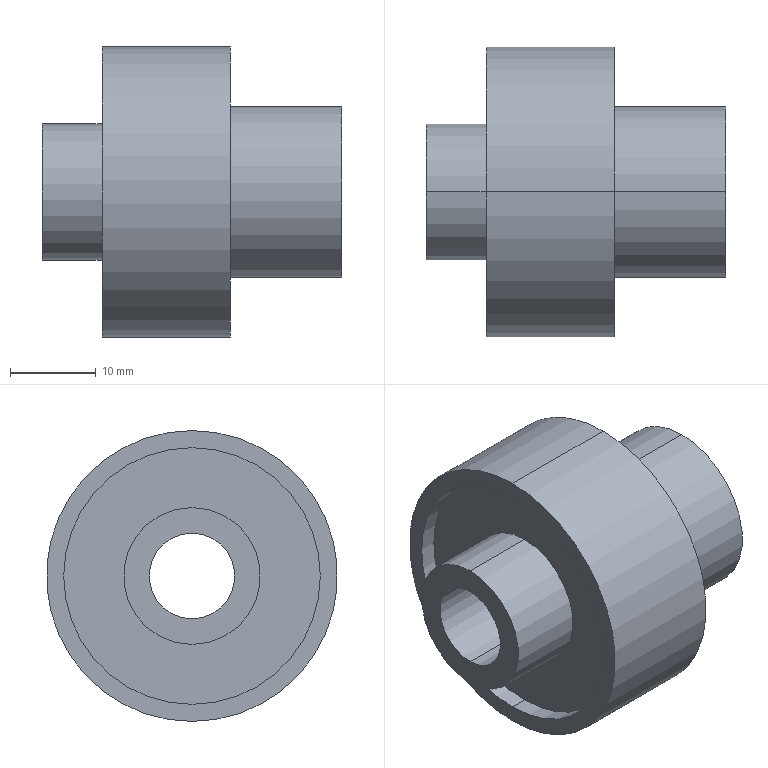Component | SolidWorks | IntermediateAxisSleeve-1 | 1 solid | 15 faces | box 35 x 34 x 34 mm | volume 15350 mm3 | cylinder 10 | plane 5 | commonest cylinder face diameters 10 x2 20 x2 34 x2 30 x2 16 x2 | material AISI 1045 Steel, Cold Drawn
build123d program:
from build123d import *


with BuildPart() as part:
    # Sketch1 → Revolve1 (revolve)
    with BuildSketch(Plane.XY, mode=Mode.PRIVATE) as revolve1_sk:
        Polygon((0, 5), (35, 5), (35, 10), (22, 10), (22, 17), (7, 17), (7, 15), (9, 15), (9, 8), (0, 8), align=None)
    revolve(revolve1_sk.sketch.rotate(Axis((-61.655, 0, 0), (1, 0, 0)), 90), axis=Axis((-61.655, 0, 0), (1, 0, 0)))


solid = part.part

# Placed as in the assembly
solid = solid.moved(Location((189.062, 15.116, 349), (0, 0, 0)))
STEP:
#1=CARTESIAN_POINT('',(8.821,0.5951,13.543));
#2=VERTEX_POINT('',#1);
#3=CARTESIAN_POINT('',(8.821,0.5951,13.937));
#4=VERTEX_POINT('',#3);
#5=CARTESIAN_POINT('',(8.821,0.5951,13.74));
#6=DIRECTION('',(-1.,0.,0.));
#7=DIRECTION('',(0.,0.,1.));
#8=AXIS2_PLACEMENT_3D('',#5,#6,#7);
#9=CIRCLE('',#8,0.1969);
#10=EDGE_CURVE('',#2,#4,#9,.T.);
#11=ORIENTED_EDGE('',*,*,#10,.F.);
#12=CARTESIAN_POINT('',(7.443,0.5951,13.543));
#13=VERTEX_POINT('',#12);
#14=CARTESIAN_POINT('',(5.016,0.5951,13.543));
#15=DIRECTION('',(-1.,0.,0.));
#16=VECTOR('',#15,39.37);
#17=LINE('',#14,#16);
#18=EDGE_CURVE('',#2,#13,#17,.T.);
#19=ORIENTED_EDGE('',*,*,#18,.T.);
#20=CARTESIAN_POINT('',(7.443,0.5951,13.937));
#21=VERTEX_POINT('',#20);
#22=CARTESIAN_POINT('',(7.443,0.5951,13.74));
#23=DIRECTION('',(-1.,0.,0.));
#24=DIRECTION('',(0.,0.,1.));
#25=AXIS2_PLACEMENT_3D('',#22,#23,#24);
#26=CIRCLE('',#25,0.1969);
#27=EDGE_CURVE('',#13,#21,#26,.T.);
#28=ORIENTED_EDGE('',*,*,#27,.T.);
#29=CARTESIAN_POINT('',(5.016,0.5951,13.937));
#30=DIRECTION('',(-1.,0.,0.));
#31=VECTOR('',#30,39.37);
#32=LINE('',#29,#31);
#33=EDGE_CURVE('',#4,#21,#32,.T.);
#34=ORIENTED_EDGE('',*,*,#33,.F.);
#35=EDGE_LOOP('',(#11,#19,#28,#34));
#36=FACE_OUTER_BOUND('',#35,.T.);
#37=CARTESIAN_POINT('',(5.016,0.5951,13.74));
#38=DIRECTION('',(-1.,0.,0.));
#39=DIRECTION('',(0.,0.,1.));
#40=AXIS2_PLACEMENT_3D('',#37,#38,#39);
#41=CYLINDRICAL_SURFACE('',#40,0.1969);
#42=ADVANCED_FACE('',(#36),#41,.F.);
#43=CARTESIAN_POINT('',(8.821,0.5951,14.134));
#44=VERTEX_POINT('',#43);
#45=CARTESIAN_POINT('',(8.821,0.5951,13.346));
#46=VERTEX_POINT('',#45);
#47=CARTESIAN_POINT('',(8.821,0.5951,13.74));
#48=DIRECTION('',(-1.,0.,0.));
#49=DIRECTION('',(0.,0.,1.));
#50=AXIS2_PLACEMENT_3D('',#47,#48,#49);
#51=CIRCLE('',#50,0.3937);
#52=EDGE_CURVE('',#44,#46,#51,.T.);
#53=ORIENTED_EDGE('',*,*,#52,.T.);
#54=CARTESIAN_POINT('',(8.31,0.5951,13.346));
#55=VERTEX_POINT('',#54);
#56=CARTESIAN_POINT('',(5.016,0.5951,13.346));
#57=DIRECTION('',(-1.,0.,0.));
#58=VECTOR('',#57,39.37);
#59=LINE('',#56,#58);
#60=EDGE_CURVE('',#46,#55,#59,.T.);
#61=ORIENTED_EDGE('',*,*,#60,.T.);
#62=CARTESIAN_POINT('',(8.31,0.5951,14.134));
#63=VERTEX_POINT('',#62);
#64=CARTESIAN_POINT('',(8.31,0.5951,13.74));
#65=DIRECTION('',(-1.,0.,0.));
#66=DIRECTION('',(0.,0.,1.));
#67=AXIS2_PLACEMENT_3D('',#64,#65,#66);
#68=CIRCLE('',#67,0.3937);
#69=EDGE_CURVE('',#63,#55,#68,.T.);
#70=ORIENTED_EDGE('',*,*,#69,.F.);
#71=CARTESIAN_POINT('',(5.016,0.5951,14.134));
#72=DIRECTION('',(-1.,0.,0.));
#73=VECTOR('',#72,39.37);
#74=LINE('',#71,#73);
#75=EDGE_CURVE('',#44,#63,#74,.T.);
#76=ORIENTED_EDGE('',*,*,#75,.F.);
#77=EDGE_LOOP('',(#53,#61,#70,#76));
#78=FACE_OUTER_BOUND('',#77,.T.);
#79=CARTESIAN_POINT('',(5.016,0.5951,13.74));
#80=DIRECTION('',(-1.,0.,0.));
#81=DIRECTION('',(0.,0.,1.));
#82=AXIS2_PLACEMENT_3D('',#79,#80,#81);
#83=CYLINDRICAL_SURFACE('',#82,0.3937);
#84=ADVANCED_FACE('',(#78),#83,.T.);
#85=CARTESIAN_POINT('',(8.31,0.5951,14.409));
#86=VERTEX_POINT('',#85);
#87=CARTESIAN_POINT('',(8.31,0.5951,13.071));
#88=VERTEX_POINT('',#87);
#89=CARTESIAN_POINT('',(8.31,0.5951,13.74));
#90=DIRECTION('',(-1.,0.,0.));
#91=DIRECTION('',(0.,0.,1.));
#92=AXIS2_PLACEMENT_3D('',#89,#90,#91);
#93=CIRCLE('',#92,0.6693);
#94=EDGE_CURVE('',#86,#88,#93,.T.);
#95=ORIENTED_EDGE('',*,*,#94,.T.);
#96=CARTESIAN_POINT('',(7.719,0.5951,13.071));
#97=VERTEX_POINT('',#96);
#98=CARTESIAN_POINT('',(5.016,0.5951,13.071));
#99=DIRECTION('',(-1.,0.,0.));
#100=VECTOR('',#99,39.37);
#101=LINE('',#98,#100);
#102=EDGE_CURVE('',#88,#97,#101,.T.);
#103=ORIENTED_EDGE('',*,*,#102,.T.);
#104=CARTESIAN_POINT('',(7.719,0.5951,14.409));
#105=VERTEX_POINT('',#104);
#106=CARTESIAN_POINT('',(7.719,0.5951,13.74));
#107=DIRECTION('',(-1.,0.,0.));
#108=DIRECTION('',(0.,0.,1.));
#109=AXIS2_PLACEMENT_3D('',#106,#107,#108);
#110=CIRCLE('',#109,0.6693);
#111=EDGE_CURVE('',#105,#97,#110,.T.);
#112=ORIENTED_EDGE('',*,*,#111,.F.);
#113=CARTESIAN_POINT('',(5.016,0.5951,14.409));
#114=DIRECTION('',(-1.,0.,0.));
#115=VECTOR('',#114,39.37);
#116=LINE('',#113,#115);
#117=EDGE_CURVE('',#86,#105,#116,.T.);
#118=ORIENTED_EDGE('',*,*,#117,.F.);
#119=EDGE_LOOP('',(#95,#103,#112,#118));
#120=FACE_OUTER_BOUND('',#119,.T.);
#121=CARTESIAN_POINT('',(5.016,0.5951,13.74));
#122=DIRECTION('',(-1.,0.,0.));
#123=DIRECTION('',(0.,0.,1.));
#124=AXIS2_PLACEMENT_3D('',#121,#122,#123);
#125=CYLINDRICAL_SURFACE('',#124,0.6693);
#126=ADVANCED_FACE('',(#120),#125,.T.);
#127=CARTESIAN_POINT('',(7.798,0.5951,13.15));
#128=VERTEX_POINT('',#127);
#129=CARTESIAN_POINT('',(7.798,0.5951,14.331));
#130=VERTEX_POINT('',#129);
#131=CARTESIAN_POINT('',(7.798,0.5951,13.74));
#132=DIRECTION('',(-1.,0.,0.));
#133=DIRECTION('',(0.,0.,1.));
#134=AXIS2_PLACEMENT_3D('',#131,#132,#133);
#135=CIRCLE('',#134,0.5906);
#136=EDGE_CURVE('',#128,#130,#135,.T.);
#137=ORIENTED_EDGE('',*,*,#136,.F.);
#138=CARTESIAN_POINT('',(7.719,0.5951,13.15));
#139=VERTEX_POINT('',#138);
#140=CARTESIAN_POINT('',(5.016,0.5951,13.15));
#141=DIRECTION('',(-1.,0.,0.));
#142=VECTOR('',#141,39.37);
#143=LINE('',#140,#142);
#144=EDGE_CURVE('',#128,#139,#143,.T.);
#145=ORIENTED_EDGE('',*,*,#144,.T.);
#146=CARTESIAN_POINT('',(7.719,0.5951,14.331));
#147=VERTEX_POINT('',#146);
#148=CARTESIAN_POINT('',(7.719,0.5951,13.74));
#149=DIRECTION('',(-1.,0.,0.));
#150=DIRECTION('',(0.,0.,1.));
#151=AXIS2_PLACEMENT_3D('',#148,#149,#150);
#152=CIRCLE('',#151,0.5906);
#153=EDGE_CURVE('',#139,#147,#152,.T.);
#154=ORIENTED_EDGE('',*,*,#153,.T.);
#155=CARTESIAN_POINT('',(5.016,0.5951,14.331));
#156=DIRECTION('',(-1.,0.,0.));
#157=VECTOR('',#156,39.37);
#158=LINE('',#155,#157);
#159=EDGE_CURVE('',#130,#147,#158,.T.);
#160=ORIENTED_EDGE('',*,*,#159,.F.);
#161=EDGE_LOOP('',(#137,#145,#154,#160));
#162=FACE_OUTER_BOUND('',#161,.T.);
#163=CARTESIAN_POINT('',(5.016,0.5951,13.74));
#164=DIRECTION('',(-1.,0.,0.));
#165=DIRECTION('',(0.,0.,1.));
#166=AXIS2_PLACEMENT_3D('',#163,#164,#165);
#167=CYLINDRICAL_SURFACE('',#166,0.5906);
#168=ADVANCED_FACE('',(#162),#167,.F.);
#169=CARTESIAN_POINT('',(7.798,0.5951,14.055));
#170=VERTEX_POINT('',#169);
#171=CARTESIAN_POINT('',(7.798,0.5951,13.425));
#172=VERTEX_POINT('',#171);
#173=CARTESIAN_POINT('',(7.798,0.5951,13.74));
#174=DIRECTION('',(-1.,0.,0.));
#175=DIRECTION('',(0.,0.,1.));
#176=AXIS2_PLACEMENT_3D('',#173,#174,#175);
#177=CIRCLE('',#176,0.315);
#178=EDGE_CURVE('',#170,#172,#177,.T.);
#179=ORIENTED_EDGE('',*,*,#178,.T.);
#180=CARTESIAN_POINT('',(7.443,0.5951,13.425));
#181=VERTEX_POINT('',#180);
#182=CARTESIAN_POINT('',(5.016,0.5951,13.425));
#183=DIRECTION('',(-1.,0.,0.));
#184=VECTOR('',#183,39.37);
#185=LINE('',#182,#184);
#186=EDGE_CURVE('',#172,#181,#185,.T.);
#187=ORIENTED_EDGE('',*,*,#186,.T.);
#188=CARTESIAN_POINT('',(7.443,0.5951,14.055));
#189=VERTEX_POINT('',#188);
#190=CARTESIAN_POINT('',(7.443,0.5951,13.74));
#191=DIRECTION('',(-1.,0.,0.));
#192=DIRECTION('',(0.,0.,1.));
#193=AXIS2_PLACEMENT_3D('',#190,#191,#192);
#194=CIRCLE('',#193,0.315);
#195=EDGE_CURVE('',#189,#181,#194,.T.);
#196=ORIENTED_EDGE('',*,*,#195,.F.);
#197=CARTESIAN_POINT('',(5.016,0.5951,14.055));
#198=DIRECTION('',(-1.,0.,0.));
#199=VECTOR('',#198,39.37);
#200=LINE('',#197,#199);
#201=EDGE_CURVE('',#170,#189,#200,.T.);
#202=ORIENTED_EDGE('',*,*,#201,.F.);
#203=EDGE_LOOP('',(#179,#187,#196,#202));
#204=FACE_OUTER_BOUND('',#203,.T.);
#205=CARTESIAN_POINT('',(5.016,0.5951,13.74));
#206=DIRECTION('',(-1.,0.,0.));
#207=DIRECTION('',(0.,0.,1.));
#208=AXIS2_PLACEMENT_3D('',#205,#206,#207);
#209=CYLINDRICAL_SURFACE('',#208,0.315);
#210=ADVANCED_FACE('',(#204),#209,.T.);
#211=CARTESIAN_POINT('',(7.443,0.5951,13.74));
#212=DIRECTION('',(-1.,0.,0.));
#213=DIRECTION('',(0.,0.,1.));
#214=AXIS2_PLACEMENT_3D('',#211,#212,#213);
#215=CIRCLE('',#214,0.1969);
#216=EDGE_CURVE('',#21,#13,#215,.T.);
#217=ORIENTED_EDGE('',*,*,#216,.F.);
#218=ORIENTED_EDGE('',*,*,#27,.F.);
#219=EDGE_LOOP('',(#217,#218));
#220=FACE_BOUND('',#219,.T.);
#221=ORIENTED_EDGE('',*,*,#195,.T.);
#222=CARTESIAN_POINT('',(7.443,0.5951,13.74));
#223=DIRECTION('',(-1.,0.,0.));
#224=DIRECTION('',(0.,0.,1.));
#225=AXIS2_PLACEMENT_3D('',#222,#223,#224);
#226=CIRCLE('',#225,0.315);
#227=EDGE_CURVE('',#181,#189,#226,.T.);
#228=ORIENTED_EDGE('',*,*,#227,.T.);
#229=EDGE_LOOP('',(#221,#228));
#230=FACE_OUTER_BOUND('',#229,.T.);
#231=CARTESIAN_POINT('',(7.443,0.792,13.74));
#232=DIRECTION('',(1.,0.,0.));
#233=DIRECTION('',(0.,0.,-1.));
#234=AXIS2_PLACEMENT_3D('',#231,#232,#233);
#235=PLANE('',#234);
#236=ADVANCED_FACE('',(#220,#230),#235,.F.);
#237=ORIENTED_EDGE('',*,*,#186,.F.);
#238=CARTESIAN_POINT('',(7.798,0.5951,13.74));
#239=DIRECTION('',(-1.,0.,0.));
#240=DIRECTION('',(0.,0.,1.));
#241=AXIS2_PLACEMENT_3D('',#238,#239,#240);
#242=CIRCLE('',#241,0.315);
#243=EDGE_CURVE('',#172,#170,#242,.T.);
#244=ORIENTED_EDGE('',*,*,#243,.T.);
#245=ORIENTED_EDGE('',*,*,#201,.T.);
#246=ORIENTED_EDGE('',*,*,#227,.F.);
#247=EDGE_LOOP('',(#237,#244,#245,#246));
#248=FACE_OUTER_BOUND('',#247,.T.);
#249=CARTESIAN_POINT('',(5.016,0.5951,13.74));
#250=DIRECTION('',(-1.,0.,0.));
#251=DIRECTION('',(0.,0.,1.));
#252=AXIS2_PLACEMENT_3D('',#249,#250,#251);
#253=CYLINDRICAL_SURFACE('',#252,0.315);
#254=ADVANCED_FACE('',(#248),#253,.T.);
#255=ORIENTED_EDGE('',*,*,#178,.F.);
#256=ORIENTED_EDGE('',*,*,#243,.F.);
#257=EDGE_LOOP('',(#255,#256));
#258=FACE_BOUND('',#257,.T.);
#259=CARTESIAN_POINT('',(7.798,0.5951,13.74));
#260=DIRECTION('',(-1.,0.,0.));
#261=DIRECTION('',(0.,0.,1.));
#262=AXIS2_PLACEMENT_3D('',#259,#260,#261);
#263=CIRCLE('',#262,0.5906);
#264=EDGE_CURVE('',#130,#128,#263,.T.);
#265=ORIENTED_EDGE('',*,*,#264,.T.);
#266=ORIENTED_EDGE('',*,*,#136,.T.);
#267=EDGE_LOOP('',(#265,#266));
#268=FACE_OUTER_BOUND('',#267,.T.);
#269=CARTESIAN_POINT('',(7.798,0.9101,13.74));
#270=DIRECTION('',(1.,0.,0.));
#271=DIRECTION('',(0.,0.,-1.));
#272=AXIS2_PLACEMENT_3D('',#269,#270,#271);
#273=PLANE('',#272);
#274=ADVANCED_FACE('',(#258,#268),#273,.F.);
#275=ORIENTED_EDGE('',*,*,#144,.F.);
#276=ORIENTED_EDGE('',*,*,#264,.F.);
#277=ORIENTED_EDGE('',*,*,#159,.T.);
#278=CARTESIAN_POINT('',(7.719,0.5951,13.74));
#279=DIRECTION('',(-1.,0.,0.));
#280=DIRECTION('',(0.,0.,1.));
#281=AXIS2_PLACEMENT_3D('',#278,#279,#280);
#282=CIRCLE('',#281,0.5906);
#283=EDGE_CURVE('',#147,#139,#282,.T.);
#284=ORIENTED_EDGE('',*,*,#283,.T.);
#285=EDGE_LOOP('',(#275,#276,#277,#284));
#286=FACE_OUTER_BOUND('',#285,.T.);
#287=CARTESIAN_POINT('',(5.016,0.5951,13.74));
#288=DIRECTION('',(-1.,0.,0.));
#289=DIRECTION('',(0.,0.,1.));
#290=AXIS2_PLACEMENT_3D('',#287,#288,#289);
#291=CYLINDRICAL_SURFACE('',#290,0.5906);
#292=ADVANCED_FACE('',(#286),#291,.F.);
#293=ORIENTED_EDGE('',*,*,#283,.F.);
#294=ORIENTED_EDGE('',*,*,#153,.F.);
#295=EDGE_LOOP('',(#293,#294));
#296=FACE_BOUND('',#295,.T.);
#297=ORIENTED_EDGE('',*,*,#111,.T.);
#298=CARTESIAN_POINT('',(7.719,0.5951,13.74));
#299=DIRECTION('',(-1.,0.,0.));
#300=DIRECTION('',(0.,0.,1.));
#301=AXIS2_PLACEMENT_3D('',#298,#299,#300);
#302=CIRCLE('',#301,0.6693);
#303=EDGE_CURVE('',#97,#105,#302,.T.);
#304=ORIENTED_EDGE('',*,*,#303,.T.);
#305=EDGE_LOOP('',(#297,#304));
#306=FACE_OUTER_BOUND('',#305,.T.);
#307=CARTESIAN_POINT('',(7.719,1.186,13.74));
#308=DIRECTION('',(1.,0.,0.));
#309=DIRECTION('',(0.,0.,-1.));
#310=AXIS2_PLACEMENT_3D('',#307,#308,#309);
#311=PLANE('',#310);
#312=ADVANCED_FACE('',(#296,#306),#311,.F.);
#313=ORIENTED_EDGE('',*,*,#102,.F.);
#314=CARTESIAN_POINT('',(8.31,0.5951,13.74));
#315=DIRECTION('',(-1.,0.,0.));
#316=DIRECTION('',(0.,0.,1.));
#317=AXIS2_PLACEMENT_3D('',#314,#315,#316);
#318=CIRCLE('',#317,0.6693);
#319=EDGE_CURVE('',#88,#86,#318,.T.);
#320=ORIENTED_EDGE('',*,*,#319,.T.);
#321=ORIENTED_EDGE('',*,*,#117,.T.);
#322=ORIENTED_EDGE('',*,*,#303,.F.);
#323=EDGE_LOOP('',(#313,#320,#321,#322));
#324=FACE_OUTER_BOUND('',#323,.T.);
#325=CARTESIAN_POINT('',(5.016,0.5951,13.74));
#326=DIRECTION('',(-1.,0.,0.));
#327=DIRECTION('',(0.,0.,1.));
#328=AXIS2_PLACEMENT_3D('',#325,#326,#327);
#329=CYLINDRICAL_SURFACE('',#328,0.6693);
#330=ADVANCED_FACE('',(#324),#329,.T.);
#331=ORIENTED_EDGE('',*,*,#94,.F.);
#332=ORIENTED_EDGE('',*,*,#319,.F.);
#333=EDGE_LOOP('',(#331,#332));
#334=FACE_OUTER_BOUND('',#333,.T.);
#335=ORIENTED_EDGE('',*,*,#69,.T.);
#336=CARTESIAN_POINT('',(8.31,0.5951,13.74));
#337=DIRECTION('',(-1.,0.,0.));
#338=DIRECTION('',(0.,0.,1.));
#339=AXIS2_PLACEMENT_3D('',#336,#337,#338);
#340=CIRCLE('',#339,0.3937);
#341=EDGE_CURVE('',#55,#63,#340,.T.);
#342=ORIENTED_EDGE('',*,*,#341,.T.);
#343=EDGE_LOOP('',(#335,#342));
#344=FACE_BOUND('',#343,.T.);
#345=CARTESIAN_POINT('',(8.31,0.9888,13.74));
#346=DIRECTION('',(-1.,0.,0.));
#347=DIRECTION('',(0.,0.,1.));
#348=AXIS2_PLACEMENT_3D('',#345,#346,#347);
#349=PLANE('',#348);
#350=ADVANCED_FACE('',(#334,#344),#349,.F.);
#351=ORIENTED_EDGE('',*,*,#60,.F.);
#352=CARTESIAN_POINT('',(8.821,0.5951,13.74));
#353=DIRECTION('',(-1.,0.,0.));
#354=DIRECTION('',(0.,0.,1.));
#355=AXIS2_PLACEMENT_3D('',#352,#353,#354);
#356=CIRCLE('',#355,0.3937);
#357=EDGE_CURVE('',#46,#44,#356,.T.);
#358=ORIENTED_EDGE('',*,*,#357,.T.);
#359=ORIENTED_EDGE('',*,*,#75,.T.);
#360=ORIENTED_EDGE('',*,*,#341,.F.);
#361=EDGE_LOOP('',(#351,#358,#359,#360));
#362=FACE_OUTER_BOUND('',#361,.T.);
#363=CARTESIAN_POINT('',(5.016,0.5951,13.74));
#364=DIRECTION('',(-1.,0.,0.));
#365=DIRECTION('',(0.,0.,1.));
#366=AXIS2_PLACEMENT_3D('',#363,#364,#365);
#367=CYLINDRICAL_SURFACE('',#366,0.3937);
#368=ADVANCED_FACE('',(#362),#367,.T.);
#369=ORIENTED_EDGE('',*,*,#52,.F.);
#370=ORIENTED_EDGE('',*,*,#357,.F.);
#371=EDGE_LOOP('',(#369,#370));
#372=FACE_OUTER_BOUND('',#371,.T.);
#373=CARTESIAN_POINT('',(8.821,0.5951,13.74));
#374=DIRECTION('',(-1.,0.,0.));
#375=DIRECTION('',(0.,0.,1.));
#376=AXIS2_PLACEMENT_3D('',#373,#374,#375);
#377=CIRCLE('',#376,0.1969);
#378=EDGE_CURVE('',#4,#2,#377,.T.);
#379=ORIENTED_EDGE('',*,*,#378,.T.);
#380=ORIENTED_EDGE('',*,*,#10,.T.);
#381=EDGE_LOOP('',(#379,#380));
#382=FACE_BOUND('',#381,.T.);
#383=CARTESIAN_POINT('',(8.821,0.9888,13.74));
#384=DIRECTION('',(-1.,0.,0.));
#385=DIRECTION('',(0.,0.,1.));
#386=AXIS2_PLACEMENT_3D('',#383,#384,#385);
#387=PLANE('',#386);
#388=ADVANCED_FACE('',(#372,#382),#387,.F.);
#389=ORIENTED_EDGE('',*,*,#18,.F.);
#390=ORIENTED_EDGE('',*,*,#378,.F.);
#391=ORIENTED_EDGE('',*,*,#33,.T.);
#392=ORIENTED_EDGE('',*,*,#216,.T.);
#393=EDGE_LOOP('',(#389,#390,#391,#392));
#394=FACE_OUTER_BOUND('',#393,.T.);
#395=CARTESIAN_POINT('',(5.016,0.5951,13.74));
#396=DIRECTION('',(-1.,0.,0.));
#397=DIRECTION('',(0.,0.,1.));
#398=AXIS2_PLACEMENT_3D('',#395,#396,#397);
#399=CYLINDRICAL_SURFACE('',#398,0.1969);
#400=ADVANCED_FACE('',(#394),#399,.F.);
#401=CLOSED_SHELL('',(#42,#84,#126,#168,#210,#236,#254,#274,#292,#312,#330,#350,#368,#388,#400));
#402=MANIFOLD_SOLID_BREP('',#401);
#403=CARTESIAN_POINT('',(0.,0.,0.));
#404=DIRECTION('',(0.,0.,1.));
#405=DIRECTION('',(1.,0.,0.));
#406=AXIS2_PLACEMENT_3D('',#403,#404,#405);
#407=(LENGTH_UNIT()NAMED_UNIT(*)SI_UNIT($,.METRE.));
#408=LENGTH_MEASURE_WITH_UNIT(LENGTH_MEASURE(0.0254),#407);
#409=DIMENSIONAL_EXPONENTS(1.,0.,0.,0.,0.,0.,0.);
#410=(CONVERSION_BASED_UNIT('',#408)LENGTH_UNIT()NAMED_UNIT(#409));
#411=UNCERTAINTY_MEASURE_WITH_UNIT(LENGTH_MEASURE(0.00001),#410,'','');
#412=(NAMED_UNIT(*)PLANE_ANGLE_UNIT()SI_UNIT($,.RADIAN.));
#413=(NAMED_UNIT(*)SI_UNIT($,.STERADIAN.)SOLID_ANGLE_UNIT());
#414=(GEOMETRIC_REPRESENTATION_CONTEXT(3)GLOBAL_UNCERTAINTY_ASSIGNED_CONTEXT((#411))GLOBAL_UNIT_ASSIGNED_CONTEXT((#410,#412,#413))REPRESENTATION_CONTEXT('',''));
#415=ADVANCED_BREP_SHAPE_REPRESENTATION('',(#402,#406),#414);
#416=COLOUR_RGB('',0.7922,0.8196,0.9333);
#417=FILL_AREA_STYLE_COLOUR('',#416);
#418=FILL_AREA_STYLE('',(#417));
#419=SURFACE_STYLE_FILL_AREA(#418);
#420=SURFACE_SIDE_STYLE('',(#419));
#421=SURFACE_STYLE_USAGE(.BOTH.,#420);
#422=PRESENTATION_STYLE_ASSIGNMENT((#421));
#423=STYLED_ITEM('',(#422),#402);
#424=(LENGTH_UNIT()NAMED_UNIT(*)SI_UNIT($,.METRE.));
#425=LENGTH_MEASURE_WITH_UNIT(LENGTH_MEASURE(0.0254),#424);
#426=DIMENSIONAL_EXPONENTS(1.,0.,0.,0.,0.,0.,0.);
#427=(CONVERSION_BASED_UNIT('',#425)LENGTH_UNIT()NAMED_UNIT(#426));
#428=UNCERTAINTY_MEASURE_WITH_UNIT(LENGTH_MEASURE(0.00001),#427,'','');
#429=(NAMED_UNIT(*)PLANE_ANGLE_UNIT()SI_UNIT($,.RADIAN.));
#430=(NAMED_UNIT(*)SI_UNIT($,.STERADIAN.)SOLID_ANGLE_UNIT());
#431=(GEOMETRIC_REPRESENTATION_CONTEXT(3)GLOBAL_UNCERTAINTY_ASSIGNED_CONTEXT((#428))GLOBAL_UNIT_ASSIGNED_CONTEXT((#427,#429,#430))REPRESENTATION_CONTEXT('',''));
#432=MECHANICAL_DESIGN_GEOMETRIC_PRESENTATION_REPRESENTATION('',(#423),#431);
#433=PRESENTATION_LAYER_ASSIGNMENT('','',(#423));